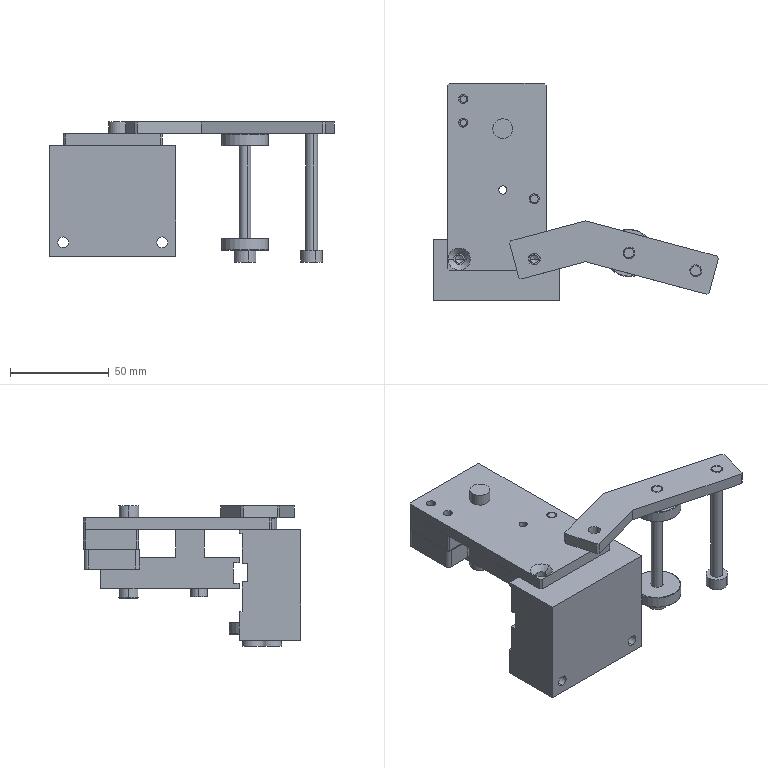Assembly | SolidWorks | mm | 13 component files | 14 solids | 201 faces | box 144.23 x 110 x 71 mm | volume 178436 mm3 | plane 90 | cylinder 83 | cone 26 | sphere 2 | commonest cylinder face diameters 10 x12 6 x10 5.5 x8 2.5 x8 3 x7 4.2 x6 4.5 x4 5 x4
Bill of materials:
BallPlungerM10X12 | 1 |  | Solid cylinder with a smaller-diameter domed (roughly hemispherical) protrusion centered on one end face.
JCT-03-01Base | 1 |  | Rectangular block with two blind holes on the top face, two through holes near the lower edge of a large side face, and a stepped recess with a central rectangular notch along one narrow side.
JCT-03-02SmallUprightPlate | 1 |  | Thin flat rectangular plate with small corner chamfers, two countersunk through holes at one end, one large through hole, and four smaller through holes.
JCT-03-03SwingBlock | 1 |  | Elongated rectangular bar with a raised rectangular boss near one end, a larger vertical through hole in the bar, a smaller through hole in the boss, and a notch/slot cut into one end face.
JCT-03-04MicroSwitchMountingBlock | 1 |  | Rectangular block with chamfered vertical corners and four vertical through holes: two larger holes along the centerline and two smaller holes at diagonally opposite corners.
JCT-03-05BentPlate | 1 |  | Flat plate of uniform thickness with an obtuse chevron (bent-outline) planform, three through holes (one at each end and one near the apex), and small corner chamfers.
JCT-03-06RetainingRing | 2 |  | Thick disc/washer-like ring with a central through bore and small chamfers on the outer edges; a small additional feature is visible intersecting the bore wall.
MicroSwitch | 1 |  | Rectangular body with rounded vertical corners, two through holes at diagonally opposite corners, and a thin angled lever arm extending from one side ending in a small cylindrical roller-like end; a rectangular recess is visible on one face.
ScrewM5X35 | 1 |  | Headed pin: short larger-diameter cylindrical head with a long smaller-diameter cylindrical shank ending in a chamfer.
ScrewM6X65 | 2 |  | Headed pin similar to a simplified fastener: short cylindrical head and a long slender cylindrical shank with a chamfered tip, more slender than unnamed part.
ThreadedRodM10X30 | 1 |  | Solid plain cylinder (dowel-like rod) with chamfered edges at both ends.
Mates:
1. concentric | JCT-03-01Base-1 face at (23.266, 3.299, 56) dir (0, 0, 1) r 2.1 | JCT-03-02SmallUprightPlate-1 face at (23.266, 3.299, 62) dir (0, 0, 1) r 2.75
2. concentric | JCT-03-01Base-1 face at (-14.734, 3.299, 56) dir (0, 0, 1) r 2.1 | JCT-03-02SmallUprightPlate-1 face at (-14.734, 3.299, 62) dir (0, 0, 1) r 2.75
3. coincident | JCT-03-01Base-1 face at (36.266, -17.701, 56) dir (0, 0, 1) | JCT-03-02SmallUprightPlate-1 face at (29.266, 92.299, 56) dir (0, 0, -1)
4. concentric | JCT-03-02SmallUprightPlate-1 face at (23.266, 33.799, 62) dir (0, 0, 1) r 2.5 | ScrewM5X35-1 face at (23.266, 33.799, -34.699) dir (0, 0, -1) r 2.5
5. coincident | JCT-03-02SmallUprightPlate-1 face at (29.266, 92.299, 62) dir (0, 0, 1) | ScrewM5X35-1 face at (23.42, 36.294, 62) dir (0, 0, 1)
6. concentric | JCT-03-02SmallUprightPlate-1 face at (7.266, 69.299, 62) dir (0, 0, 1) r 5 | BallPlungerM10X12-1 face at (7.266, 69.299, 118.996) dir (0, 0, 1) r 5
7. coincident | JCT-03-02SmallUprightPlate-1 face at (29.266, 92.299, 56) dir (0, 0, -1) | BallPlungerM10X12-1 face at (7.266, 74.299, 56) dir (0, 0, -1)
8. concentric | JCT-03-02SmallUprightPlate-1 face at (7.266, 38.299, 62) dir (0, 0, 1) r 2.1 | JCT-03-03SwingBlock-1 face at (7.266, 38.299, 26) dir (0, 0, 1) r 2.6
9. coincident | JCT-03-02SmallUprightPlate-1 face at (29.266, 92.299, 56) dir (0, 0, -1) | JCT-03-03SwingBlock-1 face at (13.266, 45.399, 56) dir (0, 0, 1)
10. parallel | JCT-03-01Base-1 face at (36.266, 11.799, 29.55) dir (0, 1, 0) | JCT-03-03SwingBlock-1 face at (13.266, 16.399, 39.1) dir (0, -1, 0)
11. concentric | JCT-03-03SwingBlock-1 face at (7.266, 69.399, 26) dir (0, 0, -1) r 5 | ThreadedRodM10X30-1 face at (7.266, 69.399, 96.869) dir (0, 0, 1) r 5
12. distance | JCT-03-03SwingBlock-1 face at (13.266, 13.399, 26) dir (0, 0, -1) | ThreadedRodM10X30-1 face at (7.266, 74.399, 21) dir (0, 0, -1)
13. concentric | JCT-03-02SmallUprightPlate-1 face at (-12.734, 84.299, 56) dir (0, 0, 1) r 2.25 | JCT-03-04MicroSwitchMountingBlock-1 face at (-12.734, 84.299, 56) dir (0, 0, 1) r 1.65
14. concentric | JCT-03-02SmallUprightPlate-1 face at (-12.734, 72.299, 56) dir (0, 0, 1) r 2.25 | JCT-03-04MicroSwitchMountingBlock-1 face at (-12.734, 72.299, 56) dir (0, 0, 1) r 1.65
15. coincident | JCT-03-02SmallUprightPlate-1 face at (29.266, 92.299, 56) dir (0, 0, -1) | JCT-03-04MicroSwitchMountingBlock-1 face at (-20.234, 64.299, 56) dir (0, 0, 1)
16. concentric | JCT-03-04MicroSwitchMountingBlock-1 face at (-7.734, 89.299, 56) dir (0, 0, 1) r 1.25 | MicroSwitch-1 face at (-7.734, 89.299, 46) dir (0, 0, -1) r 1.5
17. concentric | JCT-03-04MicroSwitchMountingBlock-1 face at (-17.734, 66.799, 56) dir (0, 0, 1) r 1.25 | MicroSwitch-1 face at (-17.734, 66.799, 46) dir (0, 0, -1) r 1.5
18. coincident | JCT-03-04MicroSwitchMountingBlock-1 face at (-20.234, 64.299, 46) dir (0, 0, -1) | MicroSwitch-1 face at (-4.734, 63.799, 46) dir (0, 0, 1)
19. concentric | JCT-03-02SmallUprightPlate-1 face at (23.266, 3.299, 62) dir (0, 0, 1) r 2.75 | JCT-03-05BentPlate-1 face at (23.266, 3.299, 62) dir (0, 0, 1) r 3
20. angle | JCT-03-02SmallUprightPlate-1 face at (29.266, 92.299, 62) dir (0, 1, 0) | JCT-03-05BentPlate-1 face at (10.501, 12.302, 68) dir (-0.2588, 0.9659, 0)
21. coincident | JCT-03-02SmallUprightPlate-1 face at (29.266, 92.299, 62) dir (0, 0, 1) | JCT-03-05BentPlate-1 face at (15.678, -7.016, 62) dir (0, 0, -1)
22. concentric | JCT-03-05BentPlate-1 face at (71.181, 6.396, 68) dir (0, 0, 1) r 3 | ScrewM6X65-1 face at (71.181, 6.396, -59.699) dir (0, 0, -1) r 3
23. coincident | JCT-03-05BentPlate-1 face at (15.678, -7.016, 68) dir (0, 0, 1) | ScrewM6X65-1 face at (68.383, 5.315, 68) dir (0, 0, 1)
24. concentric | JCT-03-05BentPlate-1 face at (104.989, -2.663, 68) dir (0, 0, 1) r 3 | ScrewM6X65-2 face at (104.989, -2.663, -59.699) dir (0, 0, -1) r 3
25. coincident | JCT-03-05BentPlate-1 face at (15.678, -7.016, 68) dir (0, 0, 1) | ScrewM6X65-2 face at (102.19, -3.744, 68) dir (0, 0, 1)
26. concentric | ScrewM6X65-1 face at (71.181, 6.396, -59.699) dir (0, 0, -1) r 3 | JCT-03-06RetainingRing-1 face at (71.181, 6.396, 62) dir (0, 0, -1) r 3.05
27. coincident | JCT-03-05BentPlate-1 face at (15.678, -7.016, 62) dir (0, 0, -1) | JCT-03-06RetainingRing-1 face at (71.181, 6.396, 62) dir (0, 0, 1)
28. concentric | ScrewM6X65-1 face at (71.181, 6.396, -59.699) dir (0, 0, -1) r 3 | JCT-03-06RetainingRing-2 face at (71.181, 6.396, 9) dir (0, 0, -1) r 3.05
29. coincident | ScrewM6X65-1 face at (66.051, 4.414, 3) dir (0, 0, 1) | JCT-03-06RetainingRing-2 face at (71.181, 6.396, 3) dir (0, 0, -1)